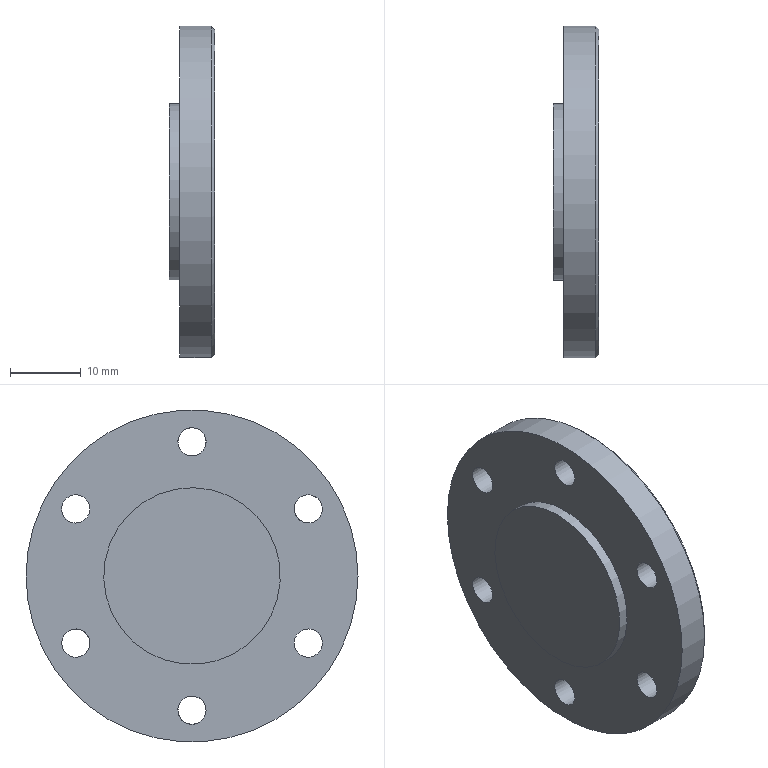Component | NX | END_CAP_1 | 1 solid | 12 faces | volume 9016 mm3 | cylinder 8 | plane 3 | cone 1 | commonest cylinder face diameters 4 x6 25 x1 47 x1